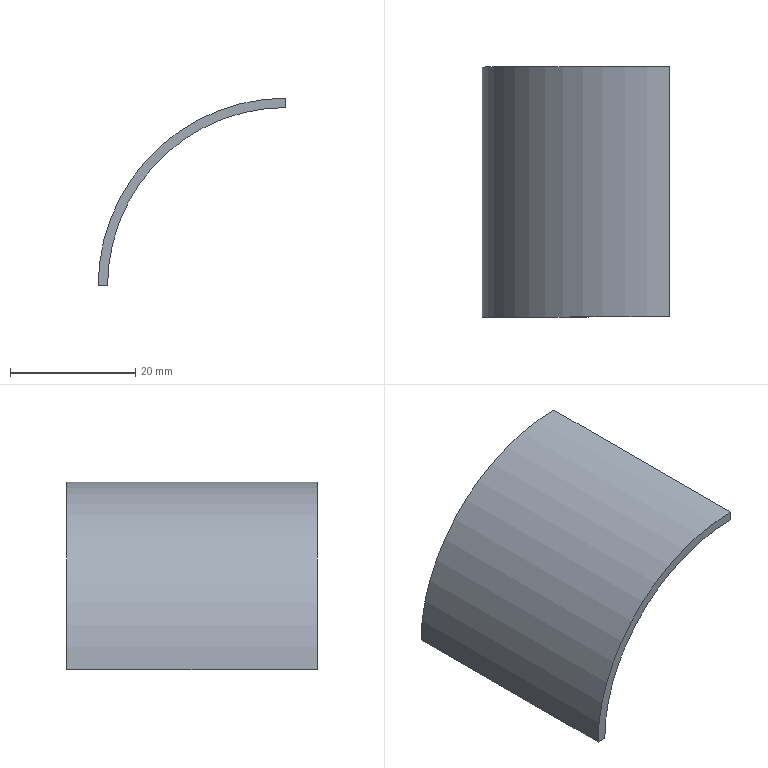Component | SolidWorks | dbj3-1_Mirror_Mirror_w12-4 | 1 solid | 6 faces | box 30 x 40 x 30 mm | volume 2757 mm3 | plane 4 | cylinder 2 | commonest cylinder face diameters 60 x1 57 x1
STEP:
#1=CARTESIAN_POINT('',(-9.843,-31.073,8.661));
#2=VERTEX_POINT('',#1);
#3=CARTESIAN_POINT('',(-8.661,-31.073,9.843));
#4=VERTEX_POINT('',#3);
#5=CARTESIAN_POINT('',(-8.661,-31.073,8.661));
#6=DIRECTION('',(-0.,1.,0.));
#7=DIRECTION('',(0.,0.,-1.));
#8=AXIS2_PLACEMENT_3D('',#5,#6,#7);
#9=CIRCLE('',#8,1.181);
#10=EDGE_CURVE('',#2,#4,#9,.T.);
#11=ORIENTED_EDGE('',*,*,#10,.T.);
#12=CARTESIAN_POINT('',(-8.661,-29.498,9.843));
#13=VERTEX_POINT('',#12);
#14=CARTESIAN_POINT('',(-8.661,-29.498,9.843));
#15=DIRECTION('',(0.,-1.,-0.));
#16=VECTOR('',#15,39.37);
#17=LINE('',#14,#16);
#18=EDGE_CURVE('',#13,#4,#17,.T.);
#19=ORIENTED_EDGE('',*,*,#18,.F.);
#20=CARTESIAN_POINT('',(-9.843,-29.498,8.661));
#21=VERTEX_POINT('',#20);
#22=CARTESIAN_POINT('',(-8.661,-29.498,8.661));
#23=DIRECTION('',(-0.,1.,0.));
#24=DIRECTION('',(0.,0.,-1.));
#25=AXIS2_PLACEMENT_3D('',#22,#23,#24);
#26=CIRCLE('',#25,1.181);
#27=EDGE_CURVE('',#21,#13,#26,.T.);
#28=ORIENTED_EDGE('',*,*,#27,.F.);
#29=CARTESIAN_POINT('',(-9.843,-29.498,8.661));
#30=DIRECTION('',(0.,-1.,-0.));
#31=VECTOR('',#30,39.37);
#32=LINE('',#29,#31);
#33=EDGE_CURVE('',#21,#2,#32,.T.);
#34=ORIENTED_EDGE('',*,*,#33,.T.);
#35=EDGE_LOOP('',(#11,#19,#28,#34));
#36=FACE_OUTER_BOUND('',#35,.T.);
#37=CARTESIAN_POINT('',(-8.661,-29.498,8.661));
#38=DIRECTION('',(0.,-1.,-0.));
#39=DIRECTION('',(0.,-0.,1.));
#40=AXIS2_PLACEMENT_3D('',#37,#38,#39);
#41=CYLINDRICAL_SURFACE('',#40,1.181);
#42=ADVANCED_FACE('',(#36),#41,.T.);
#43=CARTESIAN_POINT('',(-8.661,-31.073,9.783));
#44=VERTEX_POINT('',#43);
#45=CARTESIAN_POINT('',(-8.661,-31.073,9.783));
#46=DIRECTION('',(0.,-0.,1.));
#47=VECTOR('',#46,39.37);
#48=LINE('',#45,#47);
#49=EDGE_CURVE('',#44,#4,#48,.T.);
#50=ORIENTED_EDGE('',*,*,#49,.F.);
#51=CARTESIAN_POINT('',(-8.661,-29.498,9.783));
#52=VERTEX_POINT('',#51);
#53=CARTESIAN_POINT('',(-8.661,-29.498,9.783));
#54=DIRECTION('',(0.,-1.,-0.));
#55=VECTOR('',#54,39.37);
#56=LINE('',#53,#55);
#57=EDGE_CURVE('',#52,#44,#56,.T.);
#58=ORIENTED_EDGE('',*,*,#57,.F.);
#59=CARTESIAN_POINT('',(-8.661,-29.498,9.783));
#60=DIRECTION('',(0.,-0.,1.));
#61=VECTOR('',#60,39.37);
#62=LINE('',#59,#61);
#63=EDGE_CURVE('',#52,#13,#62,.T.);
#64=ORIENTED_EDGE('',*,*,#63,.T.);
#65=ORIENTED_EDGE('',*,*,#18,.T.);
#66=EDGE_LOOP('',(#50,#58,#64,#65));
#67=FACE_OUTER_BOUND('',#66,.T.);
#68=CARTESIAN_POINT('',(-8.661,-29.498,9.783));
#69=DIRECTION('',(1.,0.,-0.));
#70=DIRECTION('',(-0.,0.,-1.));
#71=AXIS2_PLACEMENT_3D('',#68,#69,#70);
#72=PLANE('',#71);
#73=ADVANCED_FACE('',(#67),#72,.T.);
#74=CARTESIAN_POINT('',(-9.783,-31.073,8.661));
#75=VERTEX_POINT('',#74);
#76=CARTESIAN_POINT('',(-8.661,-31.073,8.661));
#77=DIRECTION('',(-0.,1.,0.));
#78=DIRECTION('',(0.,0.,-1.));
#79=AXIS2_PLACEMENT_3D('',#76,#77,#78);
#80=CIRCLE('',#79,1.122);
#81=EDGE_CURVE('',#75,#44,#80,.T.);
#82=ORIENTED_EDGE('',*,*,#81,.F.);
#83=CARTESIAN_POINT('',(-9.783,-29.498,8.661));
#84=VERTEX_POINT('',#83);
#85=CARTESIAN_POINT('',(-9.783,-29.498,8.661));
#86=DIRECTION('',(0.,-1.,-0.));
#87=VECTOR('',#86,39.37);
#88=LINE('',#85,#87);
#89=EDGE_CURVE('',#84,#75,#88,.T.);
#90=ORIENTED_EDGE('',*,*,#89,.F.);
#91=CARTESIAN_POINT('',(-8.661,-29.498,8.661));
#92=DIRECTION('',(-0.,1.,0.));
#93=DIRECTION('',(0.,0.,-1.));
#94=AXIS2_PLACEMENT_3D('',#91,#92,#93);
#95=CIRCLE('',#94,1.122);
#96=EDGE_CURVE('',#84,#52,#95,.T.);
#97=ORIENTED_EDGE('',*,*,#96,.T.);
#98=ORIENTED_EDGE('',*,*,#57,.T.);
#99=EDGE_LOOP('',(#82,#90,#97,#98));
#100=FACE_OUTER_BOUND('',#99,.T.);
#101=CARTESIAN_POINT('',(-8.661,-29.498,8.661));
#102=DIRECTION('',(0.,-1.,-0.));
#103=DIRECTION('',(0.,-0.,1.));
#104=AXIS2_PLACEMENT_3D('',#101,#102,#103);
#105=CYLINDRICAL_SURFACE('',#104,1.122);
#106=ADVANCED_FACE('',(#100),#105,.F.);
#107=CARTESIAN_POINT('',(-9.843,-31.073,8.661));
#108=DIRECTION('',(1.,0.,-0.));
#109=VECTOR('',#108,39.37);
#110=LINE('',#107,#109);
#111=EDGE_CURVE('',#2,#75,#110,.T.);
#112=ORIENTED_EDGE('',*,*,#111,.F.);
#113=ORIENTED_EDGE('',*,*,#33,.F.);
#114=CARTESIAN_POINT('',(-9.843,-29.498,8.661));
#115=DIRECTION('',(1.,0.,-0.));
#116=VECTOR('',#115,39.37);
#117=LINE('',#114,#116);
#118=EDGE_CURVE('',#21,#84,#117,.T.);
#119=ORIENTED_EDGE('',*,*,#118,.T.);
#120=ORIENTED_EDGE('',*,*,#89,.T.);
#121=EDGE_LOOP('',(#112,#113,#119,#120));
#122=FACE_OUTER_BOUND('',#121,.T.);
#123=CARTESIAN_POINT('',(-9.843,-29.498,8.661));
#124=DIRECTION('',(-0.,0.,-1.));
#125=DIRECTION('',(-1.,-0.,0.));
#126=AXIS2_PLACEMENT_3D('',#123,#124,#125);
#127=PLANE('',#126);
#128=ADVANCED_FACE('',(#122),#127,.T.);
#129=ORIENTED_EDGE('',*,*,#27,.T.);
#130=ORIENTED_EDGE('',*,*,#63,.F.);
#131=ORIENTED_EDGE('',*,*,#96,.F.);
#132=ORIENTED_EDGE('',*,*,#118,.F.);
#133=EDGE_LOOP('',(#129,#130,#131,#132));
#134=FACE_OUTER_BOUND('',#133,.T.);
#135=CARTESIAN_POINT('',(-8.661,-29.498,8.661));
#136=DIRECTION('',(-0.,1.,0.));
#137=DIRECTION('',(-0.,0.,-1.));
#138=AXIS2_PLACEMENT_3D('',#135,#136,#137);
#139=PLANE('',#138);
#140=ADVANCED_FACE('',(#134),#139,.T.);
#141=ORIENTED_EDGE('',*,*,#10,.F.);
#142=ORIENTED_EDGE('',*,*,#111,.T.);
#143=ORIENTED_EDGE('',*,*,#81,.T.);
#144=ORIENTED_EDGE('',*,*,#49,.T.);
#145=EDGE_LOOP('',(#141,#142,#143,#144));
#146=FACE_OUTER_BOUND('',#145,.T.);
#147=CARTESIAN_POINT('',(-8.661,-31.073,8.661));
#148=DIRECTION('',(-0.,1.,0.));
#149=DIRECTION('',(-0.,0.,-1.));
#150=AXIS2_PLACEMENT_3D('',#147,#148,#149);
#151=PLANE('',#150);
#152=ADVANCED_FACE('',(#146),#151,.F.);
#153=CLOSED_SHELL('',(#42,#73,#106,#128,#140,#152));
#154=MANIFOLD_SOLID_BREP('',#153);
#155=CARTESIAN_POINT('',(0.,0.,0.));
#156=DIRECTION('',(0.,0.,1.));
#157=DIRECTION('',(1.,0.,0.));
#158=AXIS2_PLACEMENT_3D('',#155,#156,#157);
#159=(LENGTH_UNIT()NAMED_UNIT(*)SI_UNIT($,.METRE.));
#160=LENGTH_MEASURE_WITH_UNIT(LENGTH_MEASURE(0.0254),#159);
#161=DIMENSIONAL_EXPONENTS(1.,0.,0.,0.,0.,0.,0.);
#162=(CONVERSION_BASED_UNIT('',#160)LENGTH_UNIT()NAMED_UNIT(#161));
#163=UNCERTAINTY_MEASURE_WITH_UNIT(LENGTH_MEASURE(0.00001),#162,'','');
#164=(NAMED_UNIT(*)PLANE_ANGLE_UNIT()SI_UNIT($,.RADIAN.));
#165=(NAMED_UNIT(*)SI_UNIT($,.STERADIAN.)SOLID_ANGLE_UNIT());
#166=(GEOMETRIC_REPRESENTATION_CONTEXT(3)GLOBAL_UNCERTAINTY_ASSIGNED_CONTEXT((#163))GLOBAL_UNIT_ASSIGNED_CONTEXT((#162,#164,#165))REPRESENTATION_CONTEXT('',''));
#167=ADVANCED_BREP_SHAPE_REPRESENTATION('',(#154,#158),#166);
#168=COLOUR_RGB('',0.7922,0.8196,0.9333);
#169=FILL_AREA_STYLE_COLOUR('',#168);
#170=FILL_AREA_STYLE('',(#169));
#171=SURFACE_STYLE_FILL_AREA(#170);
#172=SURFACE_SIDE_STYLE('',(#171));
#173=SURFACE_STYLE_USAGE(.BOTH.,#172);
#174=PRESENTATION_STYLE_ASSIGNMENT((#173));
#175=STYLED_ITEM('',(#174),#154);
#176=PRESENTATION_LAYER_ASSIGNMENT('','',(#175));
#177=(LENGTH_UNIT()NAMED_UNIT(*)SI_UNIT($,.METRE.));
#178=LENGTH_MEASURE_WITH_UNIT(LENGTH_MEASURE(0.0254),#177);
#179=DIMENSIONAL_EXPONENTS(1.,0.,0.,0.,0.,0.,0.);
#180=(CONVERSION_BASED_UNIT('',#178)LENGTH_UNIT()NAMED_UNIT(#179));
#181=UNCERTAINTY_MEASURE_WITH_UNIT(LENGTH_MEASURE(0.00001),#180,'','');
#182=(NAMED_UNIT(*)PLANE_ANGLE_UNIT()SI_UNIT($,.RADIAN.));
#183=(NAMED_UNIT(*)SI_UNIT($,.STERADIAN.)SOLID_ANGLE_UNIT());
#184=(GEOMETRIC_REPRESENTATION_CONTEXT(3)GLOBAL_UNCERTAINTY_ASSIGNED_CONTEXT((#181))GLOBAL_UNIT_ASSIGNED_CONTEXT((#180,#182,#183))REPRESENTATION_CONTEXT('',''));
#185=MECHANICAL_DESIGN_GEOMETRIC_PRESENTATION_REPRESENTATION('',(#175),#184);